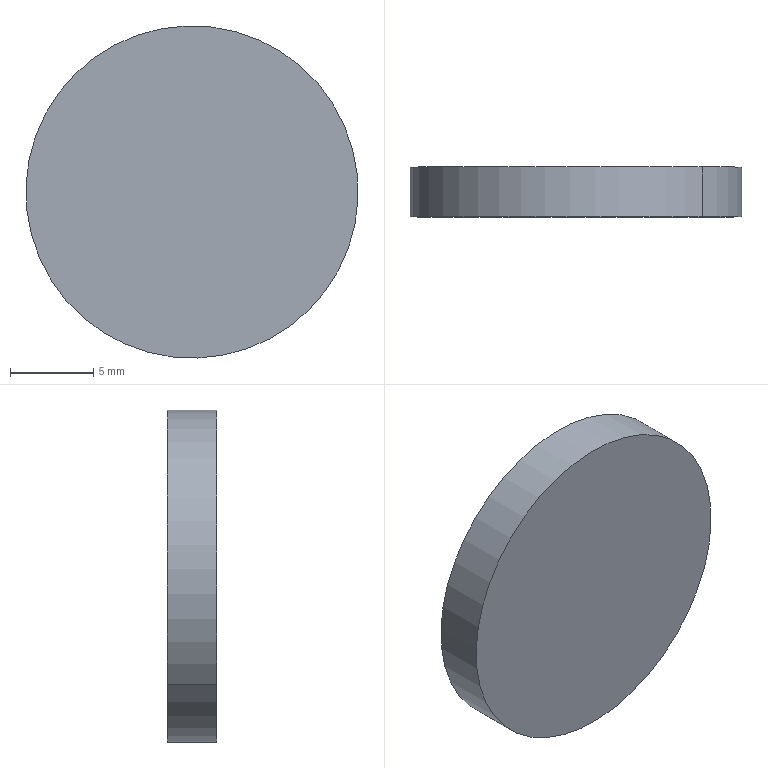Component | SolidWorks | FocusingLens-3 | 1 solid | 4 faces | box 20 x 3 x 20 mm | volume 942 mm3 | cylinder 2 | plane 2 | commonest cylinder face diameters 20 x2
build123d program:
from build123d import *

# Parameters (mm, degrees)
SKETCH1_R           = 10
BOSS_EXTRUDE1_DEPTH = 3


with BuildPart() as part:
    # Sketch1 → Boss-Extrude1 (new body)
    with BuildSketch(Plane(origin=(0, 0, 0), x_dir=(1, 0, 0), z_dir=(0, 1, 0))):
        with Locations(Location((0, 0, 0), (0, 0, 270))):
            Circle(SKETCH1_R)
    extrude(amount=BOSS_EXTRUDE1_DEPTH)


solid = part.part

# Placed as in the assembly
solid = solid.moved(Location((-45.655, 12.506, 137.094), (0, 0, 0)))
STEP:
#1=CARTESIAN_POINT('',(-1.499,0.6105,5.654));
#2=VERTEX_POINT('',#1);
#3=CARTESIAN_POINT('',(-2.096,0.6105,5.141));
#4=VERTEX_POINT('',#3);
#5=CARTESIAN_POINT('',(-1.797,0.6105,5.397));
#6=DIRECTION('',(0.,1.,0.));
#7=DIRECTION('',(0.7592,0.,0.6509));
#8=AXIS2_PLACEMENT_3D('',#5,#6,#7);
#9=CIRCLE('',#8,0.3937);
#10=EDGE_CURVE('',#2,#4,#9,.T.);
#11=ORIENTED_EDGE('',*,*,#10,.F.);
#12=CARTESIAN_POINT('',(-1.499,0.4924,5.654));
#13=VERTEX_POINT('',#12);
#14=CARTESIAN_POINT('',(-1.499,0.6105,5.654));
#15=DIRECTION('',(0.,-1.,0.));
#16=VECTOR('',#15,39.37);
#17=LINE('',#14,#16);
#18=EDGE_CURVE('',#2,#13,#17,.T.);
#19=ORIENTED_EDGE('',*,*,#18,.T.);
#20=CARTESIAN_POINT('',(-2.096,0.4924,5.141));
#21=VERTEX_POINT('',#20);
#22=CARTESIAN_POINT('',(-1.797,0.4924,5.397));
#23=DIRECTION('',(0.,1.,0.));
#24=DIRECTION('',(0.7592,0.,0.6509));
#25=AXIS2_PLACEMENT_3D('',#22,#23,#24);
#26=CIRCLE('',#25,0.3937);
#27=EDGE_CURVE('',#13,#21,#26,.T.);
#28=ORIENTED_EDGE('',*,*,#27,.T.);
#29=CARTESIAN_POINT('',(-2.096,0.6105,5.141));
#30=DIRECTION('',(0.,-1.,0.));
#31=VECTOR('',#30,39.37);
#32=LINE('',#29,#31);
#33=EDGE_CURVE('',#4,#21,#32,.T.);
#34=ORIENTED_EDGE('',*,*,#33,.F.);
#35=EDGE_LOOP('',(#11,#19,#28,#34));
#36=FACE_OUTER_BOUND('',#35,.T.);
#37=CARTESIAN_POINT('',(-1.797,0.6105,5.397));
#38=DIRECTION('',(0.,-1.,0.));
#39=DIRECTION('',(-0.7592,0.,-0.6509));
#40=AXIS2_PLACEMENT_3D('',#37,#38,#39);
#41=CYLINDRICAL_SURFACE('',#40,0.3937);
#42=ADVANCED_FACE('',(#36),#41,.T.);
#43=ORIENTED_EDGE('',*,*,#18,.F.);
#44=CARTESIAN_POINT('',(-1.797,0.6105,5.397));
#45=DIRECTION('',(0.,1.,0.));
#46=DIRECTION('',(0.7592,0.,0.6509));
#47=AXIS2_PLACEMENT_3D('',#44,#45,#46);
#48=CIRCLE('',#47,0.3937);
#49=EDGE_CURVE('',#4,#2,#48,.T.);
#50=ORIENTED_EDGE('',*,*,#49,.F.);
#51=ORIENTED_EDGE('',*,*,#33,.T.);
#52=CARTESIAN_POINT('',(-1.797,0.4924,5.397));
#53=DIRECTION('',(0.,1.,0.));
#54=DIRECTION('',(0.7592,0.,0.6509));
#55=AXIS2_PLACEMENT_3D('',#52,#53,#54);
#56=CIRCLE('',#55,0.3937);
#57=EDGE_CURVE('',#21,#13,#56,.T.);
#58=ORIENTED_EDGE('',*,*,#57,.T.);
#59=EDGE_LOOP('',(#43,#50,#51,#58));
#60=FACE_OUTER_BOUND('',#59,.T.);
#61=CARTESIAN_POINT('',(-1.797,0.6105,5.397));
#62=DIRECTION('',(0.,-1.,0.));
#63=DIRECTION('',(-0.7592,0.,-0.6509));
#64=AXIS2_PLACEMENT_3D('',#61,#62,#63);
#65=CYLINDRICAL_SURFACE('',#64,0.3937);
#66=ADVANCED_FACE('',(#60),#65,.T.);
#67=ORIENTED_EDGE('',*,*,#49,.T.);
#68=ORIENTED_EDGE('',*,*,#10,.T.);
#69=EDGE_LOOP('',(#67,#68));
#70=FACE_OUTER_BOUND('',#69,.T.);
#71=CARTESIAN_POINT('',(-1.797,0.6105,5.397));
#72=DIRECTION('',(0.,1.,0.));
#73=DIRECTION('',(0.7592,0.,0.6509));
#74=AXIS2_PLACEMENT_3D('',#71,#72,#73);
#75=PLANE('',#74);
#76=ADVANCED_FACE('',(#70),#75,.T.);
#77=ORIENTED_EDGE('',*,*,#57,.F.);
#78=ORIENTED_EDGE('',*,*,#27,.F.);
#79=EDGE_LOOP('',(#77,#78));
#80=FACE_OUTER_BOUND('',#79,.T.);
#81=CARTESIAN_POINT('',(-1.797,0.4924,5.397));
#82=DIRECTION('',(0.,1.,0.));
#83=DIRECTION('',(0.7592,0.,0.6509));
#84=AXIS2_PLACEMENT_3D('',#81,#82,#83);
#85=PLANE('',#84);
#86=ADVANCED_FACE('',(#80),#85,.F.);
#87=CLOSED_SHELL('',(#42,#66,#76,#86));
#88=MANIFOLD_SOLID_BREP('',#87);
#89=CARTESIAN_POINT('',(0.,0.,0.));
#90=DIRECTION('',(0.,0.,1.));
#91=DIRECTION('',(1.,0.,0.));
#92=AXIS2_PLACEMENT_3D('',#89,#90,#91);
#93=(LENGTH_UNIT()NAMED_UNIT(*)SI_UNIT($,.METRE.));
#94=LENGTH_MEASURE_WITH_UNIT(LENGTH_MEASURE(0.0254),#93);
#95=DIMENSIONAL_EXPONENTS(1.,0.,0.,0.,0.,0.,0.);
#96=(CONVERSION_BASED_UNIT('',#94)LENGTH_UNIT()NAMED_UNIT(#95));
#97=UNCERTAINTY_MEASURE_WITH_UNIT(LENGTH_MEASURE(0.00001),#96,'','');
#98=(NAMED_UNIT(*)PLANE_ANGLE_UNIT()SI_UNIT($,.RADIAN.));
#99=(NAMED_UNIT(*)SI_UNIT($,.STERADIAN.)SOLID_ANGLE_UNIT());
#100=(GEOMETRIC_REPRESENTATION_CONTEXT(3)GLOBAL_UNCERTAINTY_ASSIGNED_CONTEXT((#97))GLOBAL_UNIT_ASSIGNED_CONTEXT((#96,#98,#99))REPRESENTATION_CONTEXT('',''));
#101=ADVANCED_BREP_SHAPE_REPRESENTATION('',(#88,#92),#100);
#102=COLOUR_RGB('',0.7922,0.8196,0.9333);
#103=FILL_AREA_STYLE_COLOUR('',#102);
#104=FILL_AREA_STYLE('',(#103));
#105=SURFACE_STYLE_FILL_AREA(#104);
#106=SURFACE_SIDE_STYLE('',(#105));
#107=SURFACE_STYLE_USAGE(.BOTH.,#106);
#108=PRESENTATION_STYLE_ASSIGNMENT((#107));
#109=STYLED_ITEM('',(#108),#88);
#110=PRESENTATION_LAYER_ASSIGNMENT('','',(#109));
#111=(LENGTH_UNIT()NAMED_UNIT(*)SI_UNIT($,.METRE.));
#112=LENGTH_MEASURE_WITH_UNIT(LENGTH_MEASURE(0.0254),#111);
#113=DIMENSIONAL_EXPONENTS(1.,0.,0.,0.,0.,0.,0.);
#114=(CONVERSION_BASED_UNIT('',#112)LENGTH_UNIT()NAMED_UNIT(#113));
#115=UNCERTAINTY_MEASURE_WITH_UNIT(LENGTH_MEASURE(0.00001),#114,'','');
#116=(NAMED_UNIT(*)PLANE_ANGLE_UNIT()SI_UNIT($,.RADIAN.));
#117=(NAMED_UNIT(*)SI_UNIT($,.STERADIAN.)SOLID_ANGLE_UNIT());
#118=(GEOMETRIC_REPRESENTATION_CONTEXT(3)GLOBAL_UNCERTAINTY_ASSIGNED_CONTEXT((#115))GLOBAL_UNIT_ASSIGNED_CONTEXT((#114,#116,#117))REPRESENTATION_CONTEXT('',''));
#119=MECHANICAL_DESIGN_GEOMETRIC_PRESENTATION_REPRESENTATION('',(#109),#118);